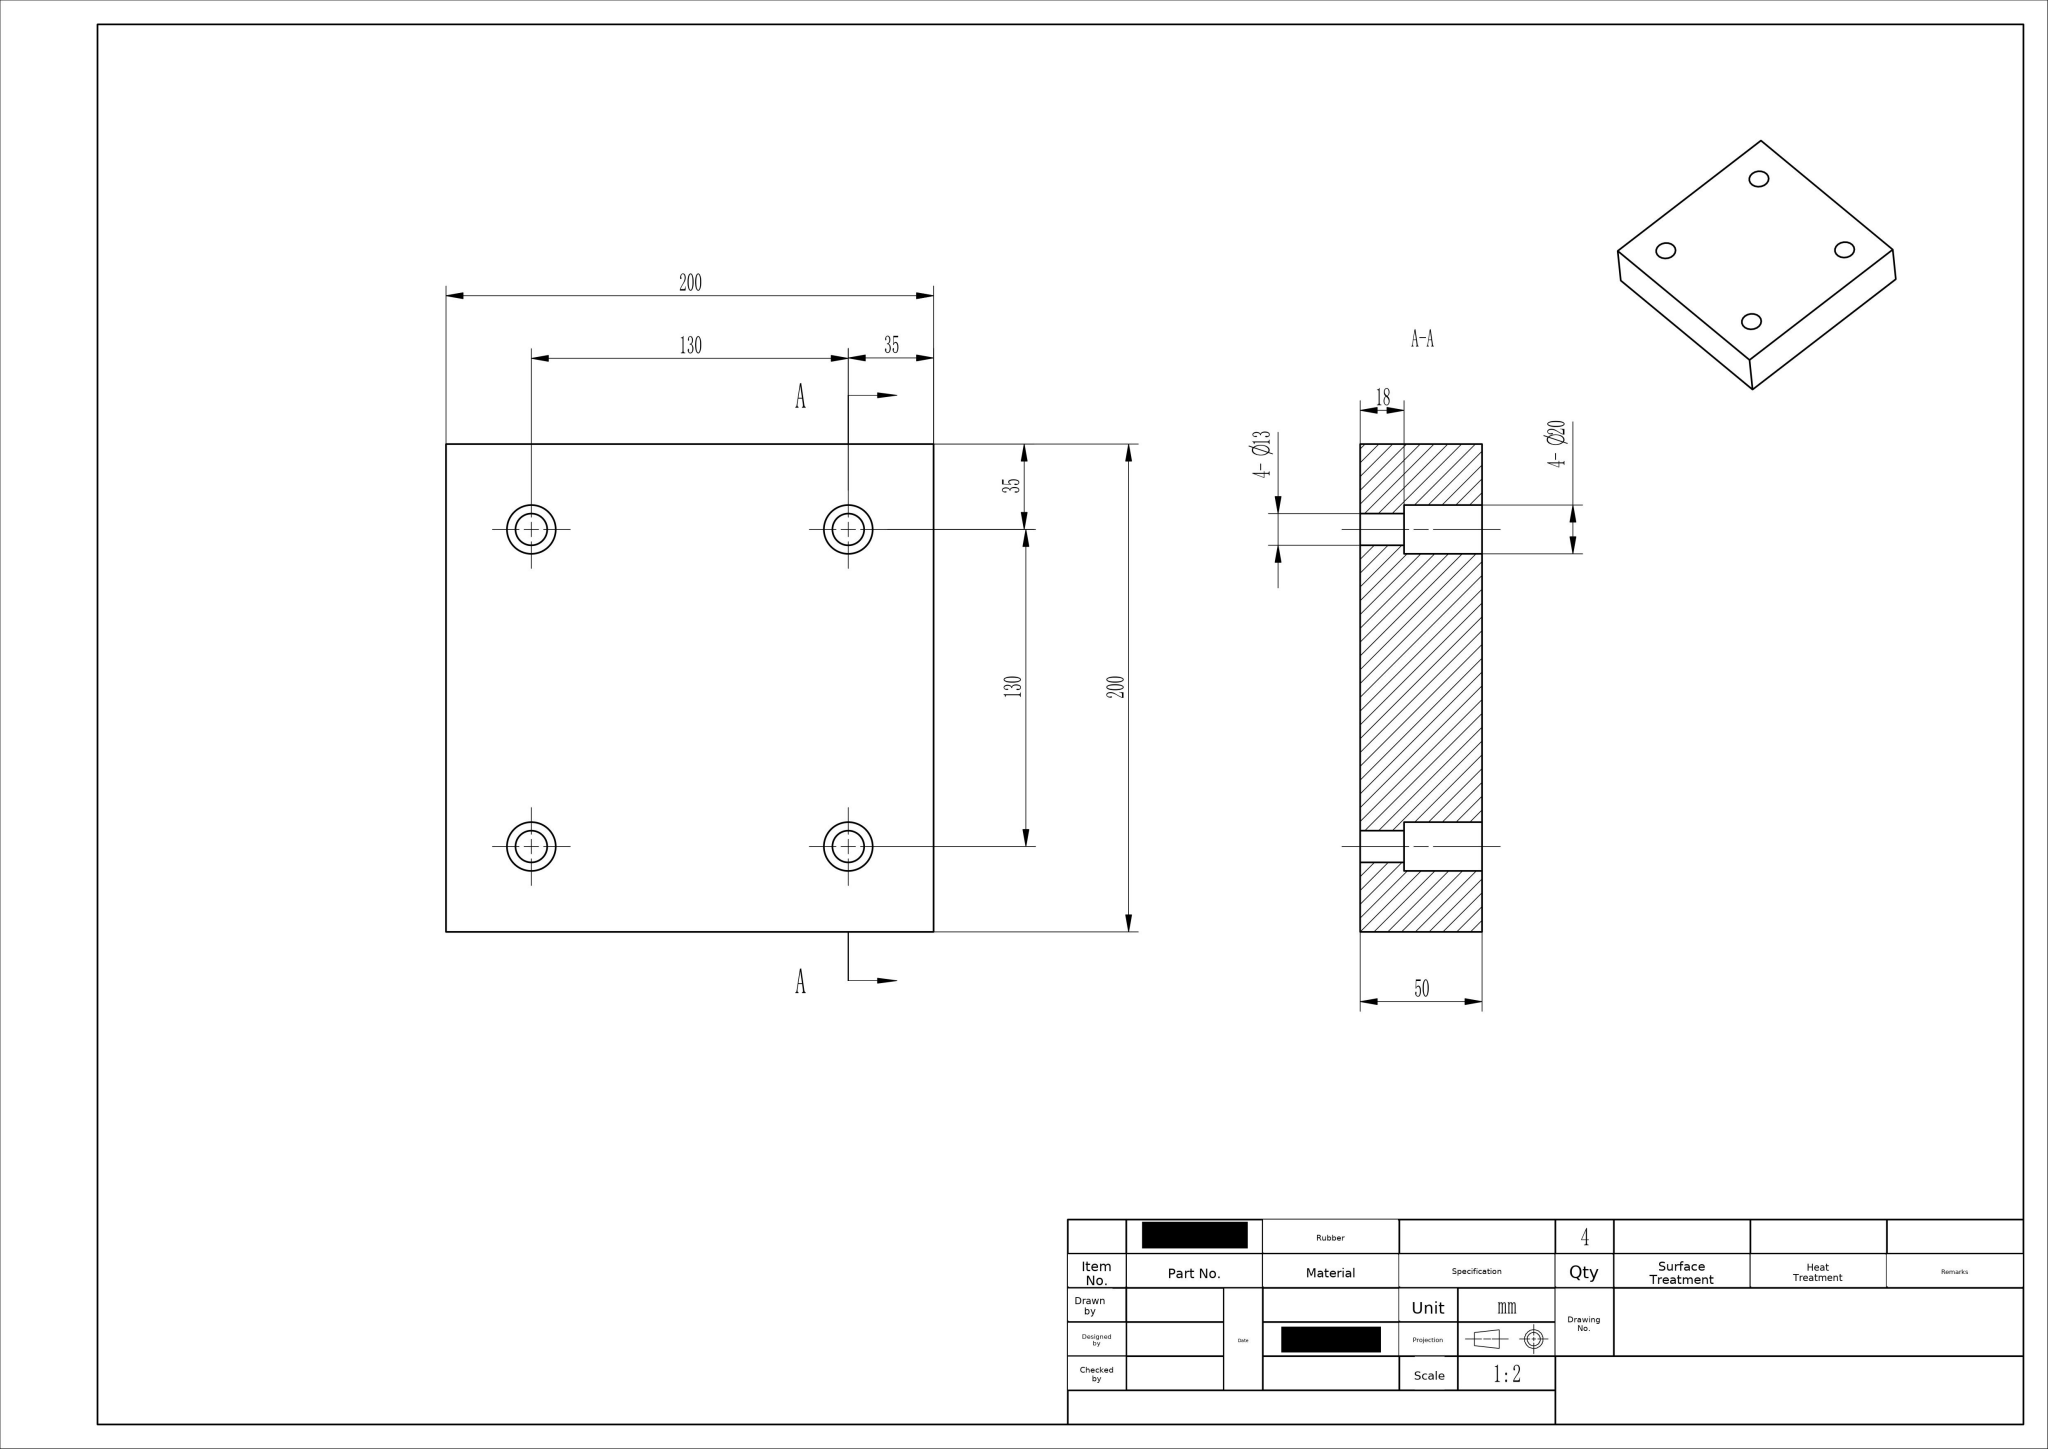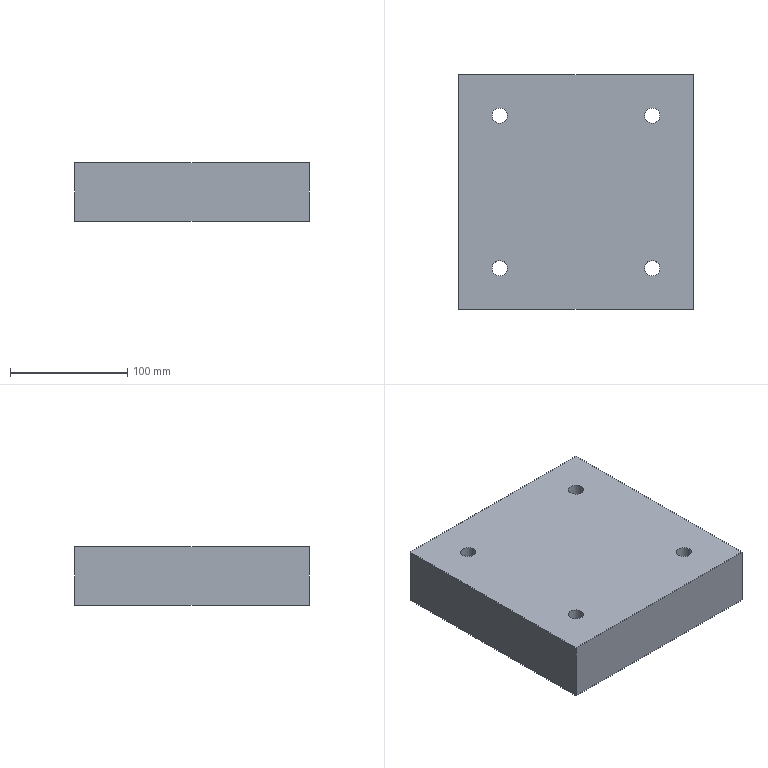Part | NX | mm | 1 solid | 18 faces | box 200 x 200 x 50 mm | volume 1950231 mm3 | plane 10 | cylinder 8 | commonest cylinder face diameters 13 x4 20 x4
STEP:
#1=CARTESIAN_POINT('',(0.,0.,0.));
#2=DIRECTION('',(0.,0.,1.));
#3=DIRECTION('',(1.,0.,0.));
#4=AXIS2_PLACEMENT_3D('',#1,#2,#3);
#5=(LENGTH_UNIT()NAMED_UNIT(*)SI_UNIT(.MILLI.,.METRE.));
#6=UNCERTAINTY_MEASURE_WITH_UNIT(LENGTH_MEASURE(0.00002),#5,'','');
#7=(NAMED_UNIT(*)PLANE_ANGLE_UNIT()SI_UNIT($,.RADIAN.));
#8=PLANE_ANGLE_MEASURE_WITH_UNIT(PLANE_ANGLE_MEASURE(0.01745),#7);
#9=DIMENSIONAL_EXPONENTS(0.,0.,0.,0.,0.,0.,0.);
#10=(CONVERSION_BASED_UNIT('',#8)NAMED_UNIT(#9)PLANE_ANGLE_UNIT());
#11=(NAMED_UNIT(*)SI_UNIT($,.STERADIAN.)SOLID_ANGLE_UNIT());
#12=(GEOMETRIC_REPRESENTATION_CONTEXT(3)GLOBAL_UNCERTAINTY_ASSIGNED_CONTEXT((#6))GLOBAL_UNIT_ASSIGNED_CONTEXT((#5,#10,#11))REPRESENTATION_CONTEXT('',''));
#13=SHAPE_REPRESENTATION('',(#4),#12);
#14=CARTESIAN_POINT('',(-100.,100.,0.));
#15=VERTEX_POINT('',#14);
#16=CARTESIAN_POINT('',(-100.,-100.,0.));
#17=VERTEX_POINT('',#16);
#18=CARTESIAN_POINT('',(-100.,100.,0.));
#19=DIRECTION('',(-0.,-1.,0.));
#20=VECTOR('',#19,1.);
#21=LINE('',#18,#20);
#22=EDGE_CURVE('',#15,#17,#21,.T.);
#23=ORIENTED_EDGE('',*,*,#22,.T.);
#24=CARTESIAN_POINT('',(-100.,-100.,50.));
#25=VERTEX_POINT('',#24);
#26=CARTESIAN_POINT('',(-100.,-100.,50.));
#27=DIRECTION('',(0.,0.,-1.));
#28=VECTOR('',#27,1.);
#29=LINE('',#26,#28);
#30=EDGE_CURVE('',#25,#17,#29,.T.);
#31=ORIENTED_EDGE('',*,*,#30,.F.);
#32=CARTESIAN_POINT('',(-100.,100.,50.));
#33=VERTEX_POINT('',#32);
#34=CARTESIAN_POINT('',(-100.,100.,50.));
#35=DIRECTION('',(-0.,-1.,0.));
#36=VECTOR('',#35,1.);
#37=LINE('',#34,#36);
#38=EDGE_CURVE('',#33,#25,#37,.T.);
#39=ORIENTED_EDGE('',*,*,#38,.F.);
#40=CARTESIAN_POINT('',(-100.,100.,50.));
#41=DIRECTION('',(0.,0.,-1.));
#42=VECTOR('',#41,1.);
#43=LINE('',#40,#42);
#44=EDGE_CURVE('',#33,#15,#43,.T.);
#45=ORIENTED_EDGE('',*,*,#44,.T.);
#46=EDGE_LOOP('',(#23,#31,#39,#45));
#47=FACE_OUTER_BOUND('',#46,.T.);
#48=CARTESIAN_POINT('',(-100.,100.,50.));
#49=DIRECTION('',(1.,-0.,0.));
#50=DIRECTION('',(0.,1.,0.));
#51=AXIS2_PLACEMENT_3D('',#48,#49,#50);
#52=PLANE('',#51);
#53=ADVANCED_FACE('',(#47),#52,.F.);
#54=CARTESIAN_POINT('',(100.,-100.,0.));
#55=VERTEX_POINT('',#54);
#56=CARTESIAN_POINT('',(-100.,-100.,0.));
#57=DIRECTION('',(1.,0.,0.));
#58=VECTOR('',#57,1.);
#59=LINE('',#56,#58);
#60=EDGE_CURVE('',#17,#55,#59,.T.);
#61=ORIENTED_EDGE('',*,*,#60,.T.);
#62=CARTESIAN_POINT('',(100.,-100.,50.));
#63=VERTEX_POINT('',#62);
#64=CARTESIAN_POINT('',(100.,-100.,50.));
#65=DIRECTION('',(0.,0.,-1.));
#66=VECTOR('',#65,1.);
#67=LINE('',#64,#66);
#68=EDGE_CURVE('',#63,#55,#67,.T.);
#69=ORIENTED_EDGE('',*,*,#68,.F.);
#70=CARTESIAN_POINT('',(-100.,-100.,50.));
#71=DIRECTION('',(1.,0.,0.));
#72=VECTOR('',#71,1.);
#73=LINE('',#70,#72);
#74=EDGE_CURVE('',#25,#63,#73,.T.);
#75=ORIENTED_EDGE('',*,*,#74,.F.);
#76=ORIENTED_EDGE('',*,*,#30,.T.);
#77=EDGE_LOOP('',(#61,#69,#75,#76));
#78=FACE_OUTER_BOUND('',#77,.T.);
#79=CARTESIAN_POINT('',(-100.,-100.,50.));
#80=DIRECTION('',(0.,1.,0.));
#81=DIRECTION('',(0.,0.,1.));
#82=AXIS2_PLACEMENT_3D('',#79,#80,#81);
#83=PLANE('',#82);
#84=ADVANCED_FACE('',(#78),#83,.F.);
#85=CARTESIAN_POINT('',(100.,100.,0.));
#86=VERTEX_POINT('',#85);
#87=CARTESIAN_POINT('',(100.,-100.,0.));
#88=DIRECTION('',(0.,1.,0.));
#89=VECTOR('',#88,1.);
#90=LINE('',#87,#89);
#91=EDGE_CURVE('',#55,#86,#90,.T.);
#92=ORIENTED_EDGE('',*,*,#91,.T.);
#93=CARTESIAN_POINT('',(100.,100.,50.));
#94=VERTEX_POINT('',#93);
#95=CARTESIAN_POINT('',(100.,100.,50.));
#96=DIRECTION('',(0.,0.,-1.));
#97=VECTOR('',#96,1.);
#98=LINE('',#95,#97);
#99=EDGE_CURVE('',#94,#86,#98,.T.);
#100=ORIENTED_EDGE('',*,*,#99,.F.);
#101=CARTESIAN_POINT('',(100.,-100.,50.));
#102=DIRECTION('',(0.,1.,0.));
#103=VECTOR('',#102,1.);
#104=LINE('',#101,#103);
#105=EDGE_CURVE('',#63,#94,#104,.T.);
#106=ORIENTED_EDGE('',*,*,#105,.F.);
#107=ORIENTED_EDGE('',*,*,#68,.T.);
#108=EDGE_LOOP('',(#92,#100,#106,#107));
#109=FACE_OUTER_BOUND('',#108,.T.);
#110=CARTESIAN_POINT('',(100.,-100.,50.));
#111=DIRECTION('',(-1.,0.,0.));
#112=DIRECTION('',(0.,0.,1.));
#113=AXIS2_PLACEMENT_3D('',#110,#111,#112);
#114=PLANE('',#113);
#115=ADVANCED_FACE('',(#109),#114,.F.);
#116=CARTESIAN_POINT('',(100.,100.,0.));
#117=DIRECTION('',(-1.,0.,0.));
#118=VECTOR('',#117,1.);
#119=LINE('',#116,#118);
#120=EDGE_CURVE('',#86,#15,#119,.T.);
#121=ORIENTED_EDGE('',*,*,#120,.T.);
#122=ORIENTED_EDGE('',*,*,#44,.F.);
#123=CARTESIAN_POINT('',(100.,100.,50.));
#124=DIRECTION('',(-1.,0.,0.));
#125=VECTOR('',#124,1.);
#126=LINE('',#123,#125);
#127=EDGE_CURVE('',#94,#33,#126,.T.);
#128=ORIENTED_EDGE('',*,*,#127,.F.);
#129=ORIENTED_EDGE('',*,*,#99,.T.);
#130=EDGE_LOOP('',(#121,#122,#128,#129));
#131=FACE_OUTER_BOUND('',#130,.T.);
#132=CARTESIAN_POINT('',(100.,100.,50.));
#133=DIRECTION('',(0.,-1.,0.));
#134=DIRECTION('',(0.,0.,-1.));
#135=AXIS2_PLACEMENT_3D('',#132,#133,#134);
#136=PLANE('',#135);
#137=ADVANCED_FACE('',(#131),#136,.F.);
#138=CARTESIAN_POINT('',(71.5,65.,50.));
#139=VERTEX_POINT('',#138);
#140=CARTESIAN_POINT('',(65.,65.,50.));
#141=DIRECTION('',(0.,0.,1.));
#142=DIRECTION('',(1.,0.,0.));
#143=AXIS2_PLACEMENT_3D('',#140,#141,#142);
#144=CIRCLE('',#143,6.5);
#145=EDGE_CURVE('',#139,#139,#144,.T.);
#146=ORIENTED_EDGE('',*,*,#145,.F.);
#147=EDGE_LOOP('',(#146));
#148=FACE_BOUND('',#147,.T.);
#149=CARTESIAN_POINT('',(71.5,-65.,50.));
#150=VERTEX_POINT('',#149);
#151=CARTESIAN_POINT('',(65.,-65.,50.));
#152=DIRECTION('',(0.,0.,1.));
#153=DIRECTION('',(1.,0.,0.));
#154=AXIS2_PLACEMENT_3D('',#151,#152,#153);
#155=CIRCLE('',#154,6.5);
#156=EDGE_CURVE('',#150,#150,#155,.T.);
#157=ORIENTED_EDGE('',*,*,#156,.F.);
#158=EDGE_LOOP('',(#157));
#159=FACE_BOUND('',#158,.T.);
#160=CARTESIAN_POINT('',(-58.5,65.,50.));
#161=VERTEX_POINT('',#160);
#162=CARTESIAN_POINT('',(-65.,65.,50.));
#163=DIRECTION('',(0.,0.,1.));
#164=DIRECTION('',(1.,0.,0.));
#165=AXIS2_PLACEMENT_3D('',#162,#163,#164);
#166=CIRCLE('',#165,6.5);
#167=EDGE_CURVE('',#161,#161,#166,.T.);
#168=ORIENTED_EDGE('',*,*,#167,.F.);
#169=EDGE_LOOP('',(#168));
#170=FACE_BOUND('',#169,.T.);
#171=CARTESIAN_POINT('',(-58.5,-65.,50.));
#172=VERTEX_POINT('',#171);
#173=CARTESIAN_POINT('',(-65.,-65.,50.));
#174=DIRECTION('',(0.,0.,1.));
#175=DIRECTION('',(1.,0.,0.));
#176=AXIS2_PLACEMENT_3D('',#173,#174,#175);
#177=CIRCLE('',#176,6.5);
#178=EDGE_CURVE('',#172,#172,#177,.T.);
#179=ORIENTED_EDGE('',*,*,#178,.F.);
#180=EDGE_LOOP('',(#179));
#181=FACE_BOUND('',#180,.T.);
#182=ORIENTED_EDGE('',*,*,#38,.T.);
#183=ORIENTED_EDGE('',*,*,#74,.T.);
#184=ORIENTED_EDGE('',*,*,#105,.T.);
#185=ORIENTED_EDGE('',*,*,#127,.T.);
#186=EDGE_LOOP('',(#182,#183,#184,#185));
#187=FACE_BOUND('',#186,.T.);
#188=CARTESIAN_POINT('',(0.,0.,50.));
#189=DIRECTION('',(0.,0.,1.));
#190=DIRECTION('',(1.,0.,0.));
#191=AXIS2_PLACEMENT_3D('',#188,#189,#190);
#192=PLANE('',#191);
#193=ADVANCED_FACE('',(#148,#159,#170,#181,#187),#192,.T.);
#194=CARTESIAN_POINT('',(75.,65.,0.));
#195=VERTEX_POINT('',#194);
#196=CARTESIAN_POINT('',(65.,65.,0.));
#197=DIRECTION('',(0.,0.,1.));
#198=DIRECTION('',(1.,0.,0.));
#199=AXIS2_PLACEMENT_3D('',#196,#197,#198);
#200=CIRCLE('',#199,10.);
#201=EDGE_CURVE('',#195,#195,#200,.T.);
#202=ORIENTED_EDGE('',*,*,#201,.T.);
#203=EDGE_LOOP('',(#202));
#204=FACE_BOUND('',#203,.T.);
#205=CARTESIAN_POINT('',(75.,-65.,0.));
#206=VERTEX_POINT('',#205);
#207=CARTESIAN_POINT('',(65.,-65.,0.));
#208=DIRECTION('',(0.,0.,1.));
#209=DIRECTION('',(1.,0.,0.));
#210=AXIS2_PLACEMENT_3D('',#207,#208,#209);
#211=CIRCLE('',#210,10.);
#212=EDGE_CURVE('',#206,#206,#211,.T.);
#213=ORIENTED_EDGE('',*,*,#212,.T.);
#214=EDGE_LOOP('',(#213));
#215=FACE_BOUND('',#214,.T.);
#216=CARTESIAN_POINT('',(-55.,65.,0.));
#217=VERTEX_POINT('',#216);
#218=CARTESIAN_POINT('',(-65.,65.,0.));
#219=DIRECTION('',(0.,0.,1.));
#220=DIRECTION('',(1.,0.,0.));
#221=AXIS2_PLACEMENT_3D('',#218,#219,#220);
#222=CIRCLE('',#221,10.);
#223=EDGE_CURVE('',#217,#217,#222,.T.);
#224=ORIENTED_EDGE('',*,*,#223,.T.);
#225=EDGE_LOOP('',(#224));
#226=FACE_BOUND('',#225,.T.);
#227=CARTESIAN_POINT('',(-55.,-65.,0.));
#228=VERTEX_POINT('',#227);
#229=CARTESIAN_POINT('',(-65.,-65.,0.));
#230=DIRECTION('',(0.,0.,1.));
#231=DIRECTION('',(1.,0.,0.));
#232=AXIS2_PLACEMENT_3D('',#229,#230,#231);
#233=CIRCLE('',#232,10.);
#234=EDGE_CURVE('',#228,#228,#233,.T.);
#235=ORIENTED_EDGE('',*,*,#234,.T.);
#236=EDGE_LOOP('',(#235));
#237=FACE_BOUND('',#236,.T.);
#238=ORIENTED_EDGE('',*,*,#22,.F.);
#239=ORIENTED_EDGE('',*,*,#120,.F.);
#240=ORIENTED_EDGE('',*,*,#91,.F.);
#241=ORIENTED_EDGE('',*,*,#60,.F.);
#242=EDGE_LOOP('',(#238,#239,#240,#241));
#243=FACE_BOUND('',#242,.T.);
#244=CARTESIAN_POINT('',(0.,0.,0.));
#245=DIRECTION('',(0.,0.,1.));
#246=DIRECTION('',(1.,0.,0.));
#247=AXIS2_PLACEMENT_3D('',#244,#245,#246);
#248=PLANE('',#247);
#249=ADVANCED_FACE('',(#204,#215,#226,#237,#243),#248,.F.);
#250=ORIENTED_EDGE('',*,*,#178,.T.);
#251=EDGE_LOOP('',(#250));
#252=FACE_BOUND('',#251,.T.);
#253=CARTESIAN_POINT('',(-58.5,-65.,32.));
#254=VERTEX_POINT('',#253);
#255=CARTESIAN_POINT('',(-65.,-65.,32.));
#256=DIRECTION('',(0.,0.,-1.));
#257=DIRECTION('',(1.,0.,0.));
#258=AXIS2_PLACEMENT_3D('',#255,#256,#257);
#259=CIRCLE('',#258,6.5);
#260=EDGE_CURVE('',#254,#254,#259,.T.);
#261=ORIENTED_EDGE('',*,*,#260,.T.);
#262=EDGE_LOOP('',(#261));
#263=FACE_BOUND('',#262,.T.);
#264=CARTESIAN_POINT('',(-65.,-65.,153.477));
#265=DIRECTION('',(0.,0.,1.));
#266=DIRECTION('',(1.,0.,0.));
#267=AXIS2_PLACEMENT_3D('',#264,#265,#266);
#268=CYLINDRICAL_SURFACE('',#267,6.5);
#269=ADVANCED_FACE('',(#252,#263),#268,.F.);
#270=ORIENTED_EDGE('',*,*,#260,.F.);
#271=EDGE_LOOP('',(#270));
#272=FACE_BOUND('',#271,.T.);
#273=CARTESIAN_POINT('',(-55.,-65.,32.));
#274=VERTEX_POINT('',#273);
#275=CARTESIAN_POINT('',(-65.,-65.,32.));
#276=DIRECTION('',(0.,0.,-1.));
#277=DIRECTION('',(1.,0.,0.));
#278=AXIS2_PLACEMENT_3D('',#275,#276,#277);
#279=CIRCLE('',#278,10.);
#280=EDGE_CURVE('',#274,#274,#279,.T.);
#281=ORIENTED_EDGE('',*,*,#280,.T.);
#282=EDGE_LOOP('',(#281));
#283=FACE_BOUND('',#282,.T.);
#284=CARTESIAN_POINT('',(-65.,-65.,32.));
#285=DIRECTION('',(0.,0.,1.));
#286=DIRECTION('',(1.,0.,0.));
#287=AXIS2_PLACEMENT_3D('',#284,#285,#286);
#288=PLANE('',#287);
#289=ADVANCED_FACE('',(#272,#283),#288,.F.);
#290=ORIENTED_EDGE('',*,*,#280,.F.);
#291=EDGE_LOOP('',(#290));
#292=FACE_BOUND('',#291,.T.);
#293=ORIENTED_EDGE('',*,*,#234,.F.);
#294=EDGE_LOOP('',(#293));
#295=FACE_BOUND('',#294,.T.);
#296=CARTESIAN_POINT('',(-65.,-65.,0.));
#297=DIRECTION('',(0.,0.,1.));
#298=DIRECTION('',(1.,0.,0.));
#299=AXIS2_PLACEMENT_3D('',#296,#297,#298);
#300=CYLINDRICAL_SURFACE('',#299,10.);
#301=ADVANCED_FACE('',(#292,#295),#300,.F.);
#302=ORIENTED_EDGE('',*,*,#167,.T.);
#303=EDGE_LOOP('',(#302));
#304=FACE_BOUND('',#303,.T.);
#305=CARTESIAN_POINT('',(-58.5,65.,32.));
#306=VERTEX_POINT('',#305);
#307=CARTESIAN_POINT('',(-65.,65.,32.));
#308=DIRECTION('',(0.,0.,-1.));
#309=DIRECTION('',(1.,0.,0.));
#310=AXIS2_PLACEMENT_3D('',#307,#308,#309);
#311=CIRCLE('',#310,6.5);
#312=EDGE_CURVE('',#306,#306,#311,.T.);
#313=ORIENTED_EDGE('',*,*,#312,.T.);
#314=EDGE_LOOP('',(#313));
#315=FACE_BOUND('',#314,.T.);
#316=CARTESIAN_POINT('',(-65.,65.,153.477));
#317=DIRECTION('',(0.,0.,1.));
#318=DIRECTION('',(1.,0.,0.));
#319=AXIS2_PLACEMENT_3D('',#316,#317,#318);
#320=CYLINDRICAL_SURFACE('',#319,6.5);
#321=ADVANCED_FACE('',(#304,#315),#320,.F.);
#322=ORIENTED_EDGE('',*,*,#312,.F.);
#323=EDGE_LOOP('',(#322));
#324=FACE_BOUND('',#323,.T.);
#325=CARTESIAN_POINT('',(-55.,65.,32.));
#326=VERTEX_POINT('',#325);
#327=CARTESIAN_POINT('',(-65.,65.,32.));
#328=DIRECTION('',(0.,0.,-1.));
#329=DIRECTION('',(1.,0.,0.));
#330=AXIS2_PLACEMENT_3D('',#327,#328,#329);
#331=CIRCLE('',#330,10.);
#332=EDGE_CURVE('',#326,#326,#331,.T.);
#333=ORIENTED_EDGE('',*,*,#332,.T.);
#334=EDGE_LOOP('',(#333));
#335=FACE_BOUND('',#334,.T.);
#336=CARTESIAN_POINT('',(-65.,65.,32.));
#337=DIRECTION('',(0.,0.,1.));
#338=DIRECTION('',(1.,0.,0.));
#339=AXIS2_PLACEMENT_3D('',#336,#337,#338);
#340=PLANE('',#339);
#341=ADVANCED_FACE('',(#324,#335),#340,.F.);
#342=ORIENTED_EDGE('',*,*,#332,.F.);
#343=EDGE_LOOP('',(#342));
#344=FACE_BOUND('',#343,.T.);
#345=ORIENTED_EDGE('',*,*,#223,.F.);
#346=EDGE_LOOP('',(#345));
#347=FACE_BOUND('',#346,.T.);
#348=CARTESIAN_POINT('',(-65.,65.,0.));
#349=DIRECTION('',(0.,0.,1.));
#350=DIRECTION('',(1.,0.,0.));
#351=AXIS2_PLACEMENT_3D('',#348,#349,#350);
#352=CYLINDRICAL_SURFACE('',#351,10.);
#353=ADVANCED_FACE('',(#344,#347),#352,.F.);
#354=ORIENTED_EDGE('',*,*,#156,.T.);
#355=EDGE_LOOP('',(#354));
#356=FACE_BOUND('',#355,.T.);
#357=CARTESIAN_POINT('',(71.5,-65.,32.));
#358=VERTEX_POINT('',#357);
#359=CARTESIAN_POINT('',(65.,-65.,32.));
#360=DIRECTION('',(0.,0.,-1.));
#361=DIRECTION('',(1.,0.,0.));
#362=AXIS2_PLACEMENT_3D('',#359,#360,#361);
#363=CIRCLE('',#362,6.5);
#364=EDGE_CURVE('',#358,#358,#363,.T.);
#365=ORIENTED_EDGE('',*,*,#364,.T.);
#366=EDGE_LOOP('',(#365));
#367=FACE_BOUND('',#366,.T.);
#368=CARTESIAN_POINT('',(65.,-65.,153.477));
#369=DIRECTION('',(0.,0.,1.));
#370=DIRECTION('',(1.,0.,0.));
#371=AXIS2_PLACEMENT_3D('',#368,#369,#370);
#372=CYLINDRICAL_SURFACE('',#371,6.5);
#373=ADVANCED_FACE('',(#356,#367),#372,.F.);
#374=ORIENTED_EDGE('',*,*,#364,.F.);
#375=EDGE_LOOP('',(#374));
#376=FACE_BOUND('',#375,.T.);
#377=CARTESIAN_POINT('',(75.,-65.,32.));
#378=VERTEX_POINT('',#377);
#379=CARTESIAN_POINT('',(65.,-65.,32.));
#380=DIRECTION('',(0.,0.,-1.));
#381=DIRECTION('',(1.,0.,0.));
#382=AXIS2_PLACEMENT_3D('',#379,#380,#381);
#383=CIRCLE('',#382,10.);
#384=EDGE_CURVE('',#378,#378,#383,.T.);
#385=ORIENTED_EDGE('',*,*,#384,.T.);
#386=EDGE_LOOP('',(#385));
#387=FACE_BOUND('',#386,.T.);
#388=CARTESIAN_POINT('',(65.,-65.,32.));
#389=DIRECTION('',(0.,0.,1.));
#390=DIRECTION('',(1.,0.,0.));
#391=AXIS2_PLACEMENT_3D('',#388,#389,#390);
#392=PLANE('',#391);
#393=ADVANCED_FACE('',(#376,#387),#392,.F.);
#394=ORIENTED_EDGE('',*,*,#384,.F.);
#395=EDGE_LOOP('',(#394));
#396=FACE_BOUND('',#395,.T.);
#397=ORIENTED_EDGE('',*,*,#212,.F.);
#398=EDGE_LOOP('',(#397));
#399=FACE_BOUND('',#398,.T.);
#400=CARTESIAN_POINT('',(65.,-65.,0.));
#401=DIRECTION('',(0.,0.,1.));
#402=DIRECTION('',(1.,0.,0.));
#403=AXIS2_PLACEMENT_3D('',#400,#401,#402);
#404=CYLINDRICAL_SURFACE('',#403,10.);
#405=ADVANCED_FACE('',(#396,#399),#404,.F.);
#406=ORIENTED_EDGE('',*,*,#145,.T.);
#407=EDGE_LOOP('',(#406));
#408=FACE_BOUND('',#407,.T.);
#409=CARTESIAN_POINT('',(71.5,65.,32.));
#410=VERTEX_POINT('',#409);
#411=CARTESIAN_POINT('',(65.,65.,32.));
#412=DIRECTION('',(0.,0.,-1.));
#413=DIRECTION('',(1.,0.,0.));
#414=AXIS2_PLACEMENT_3D('',#411,#412,#413);
#415=CIRCLE('',#414,6.5);
#416=EDGE_CURVE('',#410,#410,#415,.T.);
#417=ORIENTED_EDGE('',*,*,#416,.T.);
#418=EDGE_LOOP('',(#417));
#419=FACE_BOUND('',#418,.T.);
#420=CARTESIAN_POINT('',(65.,65.,153.477));
#421=DIRECTION('',(0.,0.,1.));
#422=DIRECTION('',(1.,0.,0.));
#423=AXIS2_PLACEMENT_3D('',#420,#421,#422);
#424=CYLINDRICAL_SURFACE('',#423,6.5);
#425=ADVANCED_FACE('',(#408,#419),#424,.F.);
#426=ORIENTED_EDGE('',*,*,#416,.F.);
#427=EDGE_LOOP('',(#426));
#428=FACE_BOUND('',#427,.T.);
#429=CARTESIAN_POINT('',(75.,65.,32.));
#430=VERTEX_POINT('',#429);
#431=CARTESIAN_POINT('',(65.,65.,32.));
#432=DIRECTION('',(0.,0.,-1.));
#433=DIRECTION('',(1.,0.,0.));
#434=AXIS2_PLACEMENT_3D('',#431,#432,#433);
#435=CIRCLE('',#434,10.);
#436=EDGE_CURVE('',#430,#430,#435,.T.);
#437=ORIENTED_EDGE('',*,*,#436,.T.);
#438=EDGE_LOOP('',(#437));
#439=FACE_BOUND('',#438,.T.);
#440=CARTESIAN_POINT('',(65.,65.,32.));
#441=DIRECTION('',(0.,0.,1.));
#442=DIRECTION('',(1.,0.,0.));
#443=AXIS2_PLACEMENT_3D('',#440,#441,#442);
#444=PLANE('',#443);
#445=ADVANCED_FACE('',(#428,#439),#444,.F.);
#446=ORIENTED_EDGE('',*,*,#436,.F.);
#447=EDGE_LOOP('',(#446));
#448=FACE_BOUND('',#447,.T.);
#449=ORIENTED_EDGE('',*,*,#201,.F.);
#450=EDGE_LOOP('',(#449));
#451=FACE_BOUND('',#450,.T.);
#452=CARTESIAN_POINT('',(65.,65.,0.));
#453=DIRECTION('',(0.,0.,1.));
#454=DIRECTION('',(1.,0.,0.));
#455=AXIS2_PLACEMENT_3D('',#452,#453,#454);
#456=CYLINDRICAL_SURFACE('',#455,10.);
#457=ADVANCED_FACE('',(#448,#451),#456,.F.);
#458=CLOSED_SHELL('',(#53,#84,#115,#137,#193,#249,#269,#289,#301,#321,#341,#353,#373,#393,#405,#425,#445,#457));
#459=MANIFOLD_SOLID_BREP('',#458);
#460=ADVANCED_BREP_SHAPE_REPRESENTATION('',(#459),#12);
#461=SHAPE_REPRESENTATION_RELATIONSHIP('','',#13,#460);
#462=PRESENTATION_LAYER_ASSIGNMENT('','',(#459));
#463=COLOUR_RGB('',0.4902,0.4902,0.4902);
#464=FILL_AREA_STYLE_COLOUR('',#463);
#465=FILL_AREA_STYLE('',(#464));
#466=SURFACE_STYLE_FILL_AREA(#465);
#467=SURFACE_SIDE_STYLE('',(#466));
#468=SURFACE_STYLE_USAGE(.BOTH.,#467);
#469=PRESENTATION_STYLE_ASSIGNMENT((#468));
#470=STYLED_ITEM('',(#469),#459);
#471=MECHANICAL_DESIGN_GEOMETRIC_PRESENTATION_REPRESENTATION('',(#470),#12);